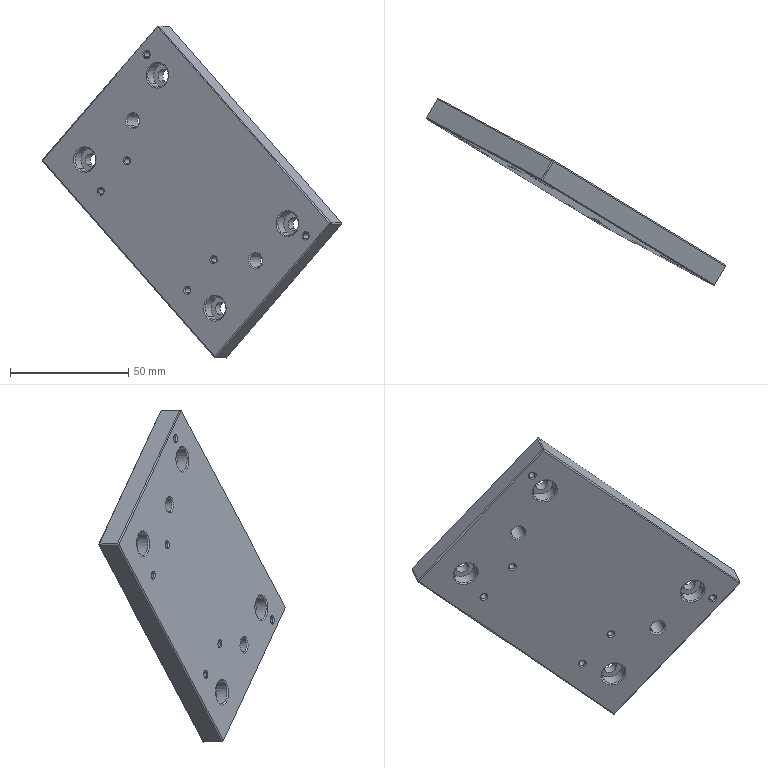Component | SolidWorks | Part7z0-123-1 | 1 solid | 102 faces | box 126.72 x 79.12 x 140.55 mm | volume 92853 mm3 | cone 48 | cylinder 32 | plane 22 | commonest cylinder face diameters 2.5 x12 10 x8 5.5 x8 6 x4
build123d program:
from build123d import *

# Parameters (mm, degrees)
SKETCH1_W                                       = 80
SKETCH1_H                                       = 120
BOSS_EXTRUDE1_DEPTH                             = 10
M3_TAPPED_HOLE1_D                               = 2.5
SIZE_MM_DOWEL_PIN_HOLE1_D                       = 6
SIZE_MM_DOWEL_PIN_HOLE1_DEPTH                   = 101.5
SIZE_MM_DOWEL_PIN_HOLE1_TIP                     = 1.803
M5_HEX_SOCKET_HEAD_CAP_SCREW_CBORE1_D           = 5.5
M5_HEX_SOCKET_HEAD_CAP_SCREW_CBORE1_CBORE_D     = 10
M5_HEX_SOCKET_HEAD_CAP_SCREW_CBORE1_CBORE_DEPTH = 5.4
CHAMFER1_SIZE                                   = 0.5
CHAMFER2_SIZE                                   = 0.5


with BuildPart() as part:
    # Sketch1 → Boss-Extrude1 (new body)
    with BuildSketch(Plane.XY):
        Rectangle(SKETCH1_W, SKETCH1_H)
    extrude(amount=BOSS_EXTRUDE1_DEPTH)

    # M3 Tapped Hole1 (through all)
    with Locations(Plane.XY.offset(10)):
        with Locations((-11, 30), (-29, 30), (-11, -30), (-29, -30), (27.5, -55), (27.5, 55)):
            Hole(M3_TAPPED_HOLE1_D / 2)

    # Size mm Dowel Pin Hole1
    with Locations(Plane.XY.offset(10)):
        with Locations((3, 40), (3, -45)):
            Hole(SIZE_MM_DOWEL_PIN_HOLE1_D / 2, depth=SIZE_MM_DOWEL_PIN_HOLE1_DEPTH)
            with Locations((0, 0, -(SIZE_MM_DOWEL_PIN_HOLE1_DEPTH + SIZE_MM_DOWEL_PIN_HOLE1_TIP / 2))):  # 118° drill point
                Cone(0, SIZE_MM_DOWEL_PIN_HOLE1_D / 2, SIZE_MM_DOWEL_PIN_HOLE1_TIP, mode=Mode.SUBTRACT)

    # M5 Hex Socket Head Cap Screw CBORE1 (through all)
    with Locations(Plane.XY.offset(10)):
        with Locations((-25, 45), (25, 45), (25, -45), (-25, -45)):
            CounterBoreHole(M5_HEX_SOCKET_HEAD_CAP_SCREW_CBORE1_D / 2, M5_HEX_SOCKET_HEAD_CAP_SCREW_CBORE1_CBORE_D / 2, M5_HEX_SOCKET_HEAD_CAP_SCREW_CBORE1_CBORE_DEPTH)

    # Chamfer1
    chamfer1_edges = [part.edges().sort_by_distance(p)[0] for p in [
        (-40, 0, 10),
        (0, -60, 10),
        (28.75, 55, 10),
        (28.75, 55, 0),
        (28.75, -55, 10),
        (28.75, -55, 0),
        (-27.75, -30, 10),
        (-27.75, -30, 0),
        (-9.75, -30, 10),
        (-9.75, -30, 0),
        (-27.75, 30, 10),
        (-27.75, 30, 0),
        (40, 0, 10),
        (-9.75, 30, 10),
        (-9.75, 30, 0),
        (0, -60, 0),
        (-40, 0, 0),
        (6, -45, 0),
        (6, -45, 10),
        (0, 60, 0),
        (6, 40, 0),
        (6, 40, 10),
        (40, 0, 0),
        (-30, -45, 10),
        (-22.25, -45, 0),
        (20, -45, 10),
        (27.75, -45, 0),
        (0, 60, 10),
        (20, 45, 10),
        (27.75, 45, 0),
        (-30, 45, 10),
        (-22.25, 45, 0),
    ]]
    chamfer(chamfer1_edges, length=CHAMFER1_SIZE)

    # Chamfer2
    chamfer2_edges = [part.edges().sort_by_distance(p)[0] for p in [
        (-40, -60, 5),
        (40, -60, 5),
        (-40, 60, 5),
        (40, 60, 5),
    ]]
    chamfer(chamfer2_edges, length=CHAMFER2_SIZE)


solid = part.part

# Placed as in the assembly
solid = solid.moved(Location((89.546, -7.244, 183.633), (88.336, -29.849, 44.87)))